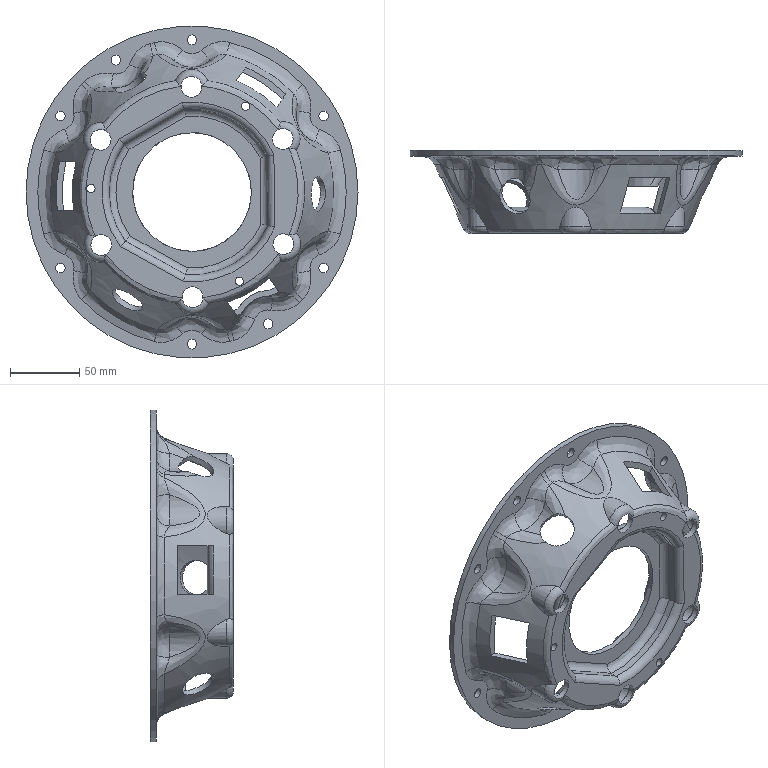Component | NX | CLUTCH_COVER | 1 solid | 217 faces | volume 240887 mm3 | spline 98 | cylinder 71 | plane 24 | torus 24 | commonest cylinder face diameters 25 x9 40 x8 48 x8 7 x8 10 x6 17 x6 15 x6 120 x3